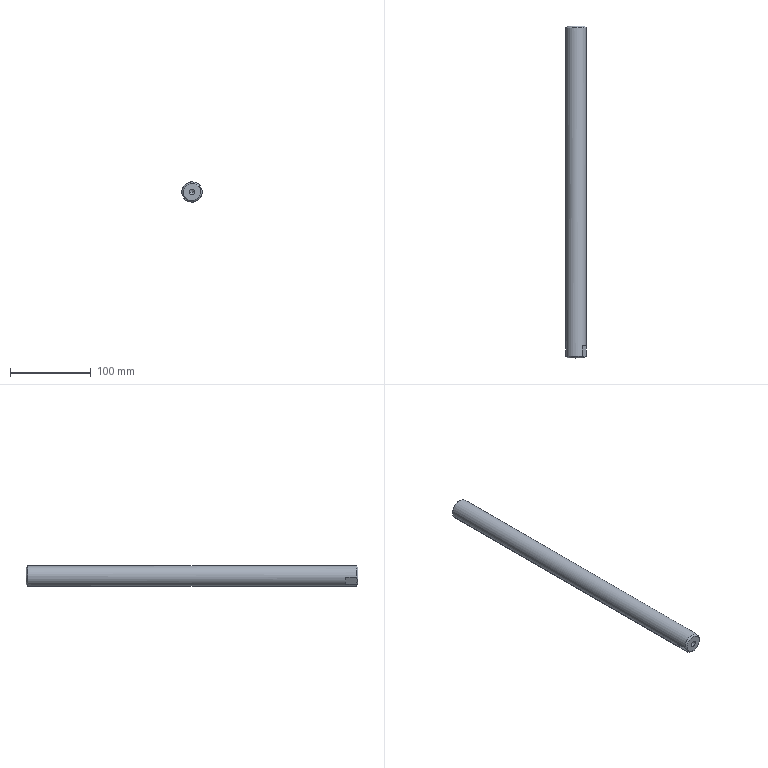Component | SolidWorks | PressingMechanism-08-2 | 1 solid | 16 faces | box 25 x 410 x 25 mm | volume 199952 mm3 | cone 6 | plane 6 | cylinder 4 | commonest cylinder face diameters 6.8 x2 25 x2
build123d program:
from build123d import *

# Parameters (mm, degrees)
SKETCH1_R             = 12.5
EXTRUDE1_DEPTH        = 410
M8_TAPPED_HOLE1_D     = 6.8
M8_TAPPED_HOLE1_DEPTH = 22.25
M8_TAPPED_HOLE1_TIP   = 2.043
CHAMFER1_SIZE         = 2
EXTRUDE2_DEPTH        = 411.381
EXTRUDE2_DEPTH_BACK   = 411.381
SKETCH6_W             = 15
SKETCH6_H             = 1


with BuildPart() as part:
    # Sketch1 → Extrude1 (new body)
    with BuildSketch(Plane(origin=(0, 0, 0), x_dir=(0, 0, -1), z_dir=(1, 0, 0))):
        with Locations(Location((0, 0, 0), (0, 0, 180))):
            Circle(SKETCH1_R)
    extrude(amount=EXTRUDE1_DEPTH)

    # M8 Tapped Hole1
    with Locations(Plane(origin=(410, 0, 0), x_dir=(0, 0, -1), z_dir=(1, 0, 0))):
        with Locations((0, 0)):
            Hole(M8_TAPPED_HOLE1_D / 2, depth=M8_TAPPED_HOLE1_DEPTH)
            with Locations((0, 0, -(M8_TAPPED_HOLE1_DEPTH + M8_TAPPED_HOLE1_TIP / 2))):  # 118° drill point
                Cone(0, M8_TAPPED_HOLE1_D / 2, M8_TAPPED_HOLE1_TIP, mode=Mode.SUBTRACT)

    # Chamfer1
    chamfer1_edges = [part.edges().sort_by_distance(p)[0] for p in [
        (0, 0, -12.5),
        (410, 0, -12.5),
    ]]
    chamfer(chamfer1_edges, length=CHAMFER1_SIZE)

    # Sketch6 → Extrude2 (cut, two sides: drawn at the far end of the back side and taken through both)
    with BuildSketch(Plane(origin=(0, 0, 0), x_dir=(1, 0, 0), z_dir=(0, 1, 0)).offset(-EXTRUDE2_DEPTH_BACK)):
        with Locations((402.5, 12)):
            Rectangle(SKETCH6_W, SKETCH6_H)
        with Locations((402.5, -12)):
            Rectangle(SKETCH6_W, SKETCH6_H)
    extrude(amount=EXTRUDE2_DEPTH + EXTRUDE2_DEPTH_BACK, mode=Mode.SUBTRACT)


solid = part.part

# Placed as in the assembly
solid = solid.moved(Location((-70, 354.5, 175), (0, 60.647, -90)))
STEP:
#1=CARTESIAN_POINT('',(-3.116,13.957,6.687));
#2=VERTEX_POINT('',#1);
#3=CARTESIAN_POINT('',(-2.396,13.957,7.092));
#4=VERTEX_POINT('',#3);
#5=CARTESIAN_POINT('',(-2.756,13.957,6.89));
#6=DIRECTION('',(0.,1.,-0.));
#7=DIRECTION('',(0.8716,0.,0.4902));
#8=AXIS2_PLACEMENT_3D('',#5,#6,#7);
#9=CIRCLE('',#8,0.4134);
#10=EDGE_CURVE('',#2,#4,#9,.T.);
#11=ORIENTED_EDGE('',*,*,#10,.F.);
#12=CARTESIAN_POINT('',(-3.185,13.878,6.649));
#13=VERTEX_POINT('',#12);
#14=CARTESIAN_POINT('',(-3.185,13.878,6.649));
#15=DIRECTION('',(-0.6163,-0.7071,-0.3466));
#16=VECTOR('',#15,39.37);
#17=LINE('',#14,#16);
#18=EDGE_CURVE('',#2,#13,#17,.T.);
#19=ORIENTED_EDGE('',*,*,#18,.T.);
#20=CARTESIAN_POINT('',(-2.327,13.878,7.131));
#21=VERTEX_POINT('',#20);
#22=CARTESIAN_POINT('',(-2.756,13.878,6.89));
#23=DIRECTION('',(-0.,-1.,0.));
#24=DIRECTION('',(0.8716,0.,0.4902));
#25=AXIS2_PLACEMENT_3D('',#22,#23,#24);
#26=CIRCLE('',#25,0.4921);
#27=EDGE_CURVE('',#21,#13,#26,.T.);
#28=ORIENTED_EDGE('',*,*,#27,.F.);
#29=CARTESIAN_POINT('',(-2.327,13.878,7.131));
#30=DIRECTION('',(0.6163,-0.7071,0.3466));
#31=VECTOR('',#30,39.37);
#32=LINE('',#29,#31);
#33=EDGE_CURVE('',#4,#21,#32,.T.);
#34=ORIENTED_EDGE('',*,*,#33,.F.);
#35=EDGE_LOOP('',(#11,#19,#28,#34));
#36=FACE_OUTER_BOUND('',#35,.T.);
#37=CARTESIAN_POINT('',(-2.756,13.878,6.89));
#38=DIRECTION('',(-0.,-1.,0.));
#39=DIRECTION('',(0.8716,0.,0.4902));
#40=AXIS2_PLACEMENT_3D('',#37,#38,#39);
#41=CONICAL_SURFACE('',#40,0.4921,0.7854);
#42=ADVANCED_FACE('',(#36),#41,.T.);
#43=CARTESIAN_POINT('',(-2.396,-2.185,7.092));
#44=VERTEX_POINT('',#43);
#45=CARTESIAN_POINT('',(-3.116,-2.185,6.687));
#46=VERTEX_POINT('',#45);
#47=CARTESIAN_POINT('',(-2.756,-2.185,6.89));
#48=DIRECTION('',(-0.,-1.,0.));
#49=DIRECTION('',(0.8716,0.,0.4902));
#50=AXIS2_PLACEMENT_3D('',#47,#48,#49);
#51=CIRCLE('',#50,0.4134);
#52=EDGE_CURVE('',#44,#46,#51,.T.);
#53=ORIENTED_EDGE('',*,*,#52,.F.);
#54=CARTESIAN_POINT('',(-2.361,-2.146,7.112));
#55=VERTEX_POINT('',#54);
#56=CARTESIAN_POINT('',(-2.396,-2.185,7.092));
#57=DIRECTION('',(0.6163,0.7071,0.3466));
#58=VECTOR('',#57,39.37);
#59=LINE('',#56,#58);
#60=EDGE_CURVE('',#44,#55,#59,.T.);
#61=ORIENTED_EDGE('',*,*,#60,.T.);
#62=CARTESIAN_POINT('',(-2.456,-2.106,7.28));
#63=VERTEX_POINT('',#62);
#64=CARTESIAN_POINT('',(-2.456,-2.106,7.28));
#65=CARTESIAN_POINT('',(-2.448,-2.112,7.266));
#66=CARTESIAN_POINT('',(-2.441,-2.118,7.253));
#67=CARTESIAN_POINT('',(-2.425,-2.128,7.225));
#68=CARTESIAN_POINT('',(-2.417,-2.132,7.211));
#69=CARTESIAN_POINT('',(-2.402,-2.139,7.183));
#70=CARTESIAN_POINT('',(-2.394,-2.141,7.169));
#71=CARTESIAN_POINT('',(-2.378,-2.145,7.141));
#72=CARTESIAN_POINT('',(-2.369,-2.146,7.126));
#73=CARTESIAN_POINT('',(-2.361,-2.146,7.112));
#74=B_SPLINE_CURVE_WITH_KNOTS('',3,(#64,#65,#66,#67,#68,#69,#70,#71,#72,#73),.UNSPECIFIED.,.F.,.F.,(4,2,2,2,4),(0.009607,0.01085,0.01209,0.01333,0.01458),.UNSPECIFIED.);
#75=EDGE_CURVE('',#63,#55,#74,.T.);
#76=ORIENTED_EDGE('',*,*,#75,.F.);
#77=CARTESIAN_POINT('',(-3.245,-2.106,6.836));
#78=VERTEX_POINT('',#77);
#79=CARTESIAN_POINT('',(-2.756,-2.106,6.89));
#80=DIRECTION('',(0.,1.,-0.));
#81=DIRECTION('',(0.8716,0.,0.4902));
#82=AXIS2_PLACEMENT_3D('',#79,#80,#81);
#83=CIRCLE('',#82,0.4921);
#84=EDGE_CURVE('',#78,#63,#83,.T.);
#85=ORIENTED_EDGE('',*,*,#84,.F.);
#86=CARTESIAN_POINT('',(-3.151,-2.146,6.668));
#87=VERTEX_POINT('',#86);
#88=CARTESIAN_POINT('',(-3.151,-2.146,6.668));
#89=CARTESIAN_POINT('',(-3.159,-2.146,6.682));
#90=CARTESIAN_POINT('',(-3.167,-2.145,6.697));
#91=CARTESIAN_POINT('',(-3.183,-2.141,6.725));
#92=CARTESIAN_POINT('',(-3.191,-2.139,6.74));
#93=CARTESIAN_POINT('',(-3.207,-2.132,6.768));
#94=CARTESIAN_POINT('',(-3.214,-2.128,6.781));
#95=CARTESIAN_POINT('',(-3.23,-2.118,6.809));
#96=CARTESIAN_POINT('',(-3.238,-2.112,6.823));
#97=CARTESIAN_POINT('',(-3.245,-2.106,6.836));
#98=B_SPLINE_CURVE_WITH_KNOTS('',3,(#88,#89,#90,#91,#92,#93,#94,#95,#96,#97),.UNSPECIFIED.,.F.,.F.,(4,2,2,2,4),(0.03511,0.03635,0.03759,0.03883,0.04007),.UNSPECIFIED.);
#99=EDGE_CURVE('',#87,#78,#98,.T.);
#100=ORIENTED_EDGE('',*,*,#99,.F.);
#101=CARTESIAN_POINT('',(-3.116,-2.185,6.687));
#102=DIRECTION('',(-0.6163,0.7071,-0.3466));
#103=VECTOR('',#102,39.37);
#104=LINE('',#101,#103);
#105=EDGE_CURVE('',#46,#87,#104,.T.);
#106=ORIENTED_EDGE('',*,*,#105,.F.);
#107=EDGE_LOOP('',(#53,#61,#76,#85,#100,#106));
#108=FACE_OUTER_BOUND('',#107,.T.);
#109=CARTESIAN_POINT('',(-2.756,-2.185,6.89));
#110=DIRECTION('',(0.,1.,-0.));
#111=DIRECTION('',(-0.8716,0.,-0.4902));
#112=AXIS2_PLACEMENT_3D('',#109,#110,#111);
#113=CONICAL_SURFACE('',#112,0.4134,0.7854);
#114=ADVANCED_FACE('',(#108),#113,.T.);
#115=CARTESIAN_POINT('',(-2.873,-1.309,6.824));
#116=VERTEX_POINT('',#115);
#117=CARTESIAN_POINT('',(-2.639,-1.309,6.955));
#118=VERTEX_POINT('',#117);
#119=CARTESIAN_POINT('',(-2.756,-1.309,6.89));
#120=DIRECTION('',(-0.,-1.,0.));
#121=DIRECTION('',(0.8716,0.,0.4902));
#122=AXIS2_PLACEMENT_3D('',#119,#120,#121);
#123=CIRCLE('',#122,0.1339);
#124=EDGE_CURVE('',#116,#118,#123,.T.);
#125=ORIENTED_EDGE('',*,*,#124,.F.);
#126=CARTESIAN_POINT('',(-2.873,-2.185,6.824));
#127=VERTEX_POINT('',#126);
#128=CARTESIAN_POINT('',(-2.873,-2.185,6.824));
#129=DIRECTION('',(-0.,-1.,0.));
#130=VECTOR('',#129,39.37);
#131=LINE('',#128,#130);
#132=EDGE_CURVE('',#116,#127,#131,.T.);
#133=ORIENTED_EDGE('',*,*,#132,.T.);
#134=CARTESIAN_POINT('',(-2.639,-2.185,6.955));
#135=VERTEX_POINT('',#134);
#136=CARTESIAN_POINT('',(-2.756,-2.185,6.89));
#137=DIRECTION('',(-0.,-1.,0.));
#138=DIRECTION('',(0.8716,0.,0.4902));
#139=AXIS2_PLACEMENT_3D('',#136,#137,#138);
#140=CIRCLE('',#139,0.1339);
#141=EDGE_CURVE('',#127,#135,#140,.T.);
#142=ORIENTED_EDGE('',*,*,#141,.T.);
#143=CARTESIAN_POINT('',(-2.639,-2.185,6.955));
#144=DIRECTION('',(-0.,-1.,0.));
#145=VECTOR('',#144,39.37);
#146=LINE('',#143,#145);
#147=EDGE_CURVE('',#118,#135,#146,.T.);
#148=ORIENTED_EDGE('',*,*,#147,.F.);
#149=EDGE_LOOP('',(#125,#133,#142,#148));
#150=FACE_OUTER_BOUND('',#149,.T.);
#151=CARTESIAN_POINT('',(-2.756,-2.185,6.89));
#152=DIRECTION('',(-0.,-1.,0.));
#153=DIRECTION('',(0.8716,0.,0.4902));
#154=AXIS2_PLACEMENT_3D('',#151,#152,#153);
#155=CYLINDRICAL_SURFACE('',#154,0.1339);
#156=ADVANCED_FACE('',(#150),#155,.F.);
#157=CARTESIAN_POINT('',(-2.756,-1.229,6.89));
#158=VERTEX_POINT('',#157);
#159=CARTESIAN_POINT('',(-2.639,-1.309,6.955));
#160=DIRECTION('',(0.7471,-0.515,0.4202));
#161=VECTOR('',#160,39.37);
#162=LINE('',#159,#161);
#163=EDGE_CURVE('',#158,#118,#162,.T.);
#164=ORIENTED_EDGE('',*,*,#163,.F.);
#165=CARTESIAN_POINT('',(-2.873,-1.309,6.824));
#166=DIRECTION('',(-0.7471,-0.515,-0.4202));
#167=VECTOR('',#166,39.37);
#168=LINE('',#165,#167);
#169=EDGE_CURVE('',#158,#116,#168,.T.);
#170=ORIENTED_EDGE('',*,*,#169,.T.);
#171=ORIENTED_EDGE('',*,*,#124,.T.);
#172=EDGE_LOOP('',(#164,#170,#171));
#173=FACE_OUTER_BOUND('',#172,.T.);
#174=CARTESIAN_POINT('',(-2.756,-1.309,6.89));
#175=DIRECTION('',(-0.,-1.,0.));
#176=DIRECTION('',(0.8716,0.,0.4902));
#177=AXIS2_PLACEMENT_3D('',#174,#175,#176);
#178=CONICAL_SURFACE('',#177,0.1339,1.03);
#179=ADVANCED_FACE('',(#173),#178,.F.);
#180=CARTESIAN_POINT('',(-2.456,-1.594,7.28));
#181=VERTEX_POINT('',#180);
#182=CARTESIAN_POINT('',(-2.327,-1.594,7.131));
#183=VERTEX_POINT('',#182);
#184=CARTESIAN_POINT('',(-2.756,-1.594,6.89));
#185=DIRECTION('',(0.,1.,-0.));
#186=DIRECTION('',(-0.8716,-0.,-0.4902));
#187=AXIS2_PLACEMENT_3D('',#184,#185,#186);
#188=CIRCLE('',#187,0.4921);
#189=EDGE_CURVE('',#181,#183,#188,.T.);
#190=ORIENTED_EDGE('',*,*,#189,.T.);
#191=CARTESIAN_POINT('',(-2.327,-2.185,7.131));
#192=DIRECTION('',(0.,1.,-0.));
#193=VECTOR('',#192,39.37);
#194=LINE('',#191,#193);
#195=EDGE_CURVE('',#183,#21,#194,.T.);
#196=ORIENTED_EDGE('',*,*,#195,.T.);
#197=ORIENTED_EDGE('',*,*,#27,.T.);
#198=CARTESIAN_POINT('',(-3.185,-1.594,6.649));
#199=VERTEX_POINT('',#198);
#200=CARTESIAN_POINT('',(-3.185,-2.185,6.649));
#201=DIRECTION('',(0.,1.,-0.));
#202=VECTOR('',#201,39.37);
#203=LINE('',#200,#202);
#204=EDGE_CURVE('',#199,#13,#203,.T.);
#205=ORIENTED_EDGE('',*,*,#204,.F.);
#206=CARTESIAN_POINT('',(-3.245,-1.594,6.836));
#207=VERTEX_POINT('',#206);
#208=CARTESIAN_POINT('',(-2.756,-1.594,6.89));
#209=DIRECTION('',(0.,1.,-0.));
#210=DIRECTION('',(-0.8716,-0.,-0.4902));
#211=AXIS2_PLACEMENT_3D('',#208,#209,#210);
#212=CIRCLE('',#211,0.4921);
#213=EDGE_CURVE('',#199,#207,#212,.T.);
#214=ORIENTED_EDGE('',*,*,#213,.T.);
#215=CARTESIAN_POINT('',(-3.245,-2.185,6.836));
#216=DIRECTION('',(-0.,-1.,0.));
#217=VECTOR('',#216,39.37);
#218=LINE('',#215,#217);
#219=EDGE_CURVE('',#207,#78,#218,.T.);
#220=ORIENTED_EDGE('',*,*,#219,.T.);
#221=ORIENTED_EDGE('',*,*,#84,.T.);
#222=CARTESIAN_POINT('',(-2.456,-2.185,7.28));
#223=DIRECTION('',(0.,1.,-0.));
#224=VECTOR('',#223,39.37);
#225=LINE('',#222,#224);
#226=EDGE_CURVE('',#63,#181,#225,.T.);
#227=ORIENTED_EDGE('',*,*,#226,.T.);
#228=EDGE_LOOP('',(#190,#196,#197,#205,#214,#220,#221,#227));
#229=FACE_OUTER_BOUND('',#228,.T.);
#230=CARTESIAN_POINT('',(-2.756,-2.185,6.89));
#231=DIRECTION('',(0.,1.,-0.));
#232=DIRECTION('',(-0.8716,-0.,-0.4902));
#233=AXIS2_PLACEMENT_3D('',#230,#231,#232);
#234=CYLINDRICAL_SURFACE('',#233,0.4921);
#235=ADVANCED_FACE('',(#229),#234,.T.);
#236=ORIENTED_EDGE('',*,*,#195,.F.);
#237=CARTESIAN_POINT('',(-2.267,-1.594,6.944));
#238=VERTEX_POINT('',#237);
#239=CARTESIAN_POINT('',(-2.756,-1.594,6.89));
#240=DIRECTION('',(0.,1.,-0.));
#241=DIRECTION('',(-0.8716,-0.,-0.4902));
#242=AXIS2_PLACEMENT_3D('',#239,#240,#241);
#243=CIRCLE('',#242,0.4921);
#244=EDGE_CURVE('',#183,#238,#243,.T.);
#245=ORIENTED_EDGE('',*,*,#244,.T.);
#246=CARTESIAN_POINT('',(-2.267,-2.106,6.944));
#247=VERTEX_POINT('',#246);
#248=CARTESIAN_POINT('',(-2.267,-2.185,6.944));
#249=DIRECTION('',(-0.,-1.,0.));
#250=VECTOR('',#249,39.37);
#251=LINE('',#248,#250);
#252=EDGE_CURVE('',#238,#247,#251,.T.);
#253=ORIENTED_EDGE('',*,*,#252,.T.);
#254=CARTESIAN_POINT('',(-3.056,-2.106,6.5));
#255=VERTEX_POINT('',#254);
#256=CARTESIAN_POINT('',(-2.756,-2.106,6.89));
#257=DIRECTION('',(0.,1.,-0.));
#258=DIRECTION('',(0.8716,0.,0.4902));
#259=AXIS2_PLACEMENT_3D('',#256,#257,#258);
#260=CIRCLE('',#259,0.4921);
#261=EDGE_CURVE('',#247,#255,#260,.T.);
#262=ORIENTED_EDGE('',*,*,#261,.T.);
#263=CARTESIAN_POINT('',(-3.056,-1.594,6.5));
#264=VERTEX_POINT('',#263);
#265=CARTESIAN_POINT('',(-3.056,-2.185,6.5));
#266=DIRECTION('',(0.,1.,-0.));
#267=VECTOR('',#266,39.37);
#268=LINE('',#265,#267);
#269=EDGE_CURVE('',#255,#264,#268,.T.);
#270=ORIENTED_EDGE('',*,*,#269,.T.);
#271=CARTESIAN_POINT('',(-2.756,-1.594,6.89));
#272=DIRECTION('',(0.,1.,-0.));
#273=DIRECTION('',(-0.8716,-0.,-0.4902));
#274=AXIS2_PLACEMENT_3D('',#271,#272,#273);
#275=CIRCLE('',#274,0.4921);
#276=EDGE_CURVE('',#264,#199,#275,.T.);
#277=ORIENTED_EDGE('',*,*,#276,.T.);
#278=ORIENTED_EDGE('',*,*,#204,.T.);
#279=CARTESIAN_POINT('',(-2.756,13.878,6.89));
#280=DIRECTION('',(-0.,-1.,0.));
#281=DIRECTION('',(0.8716,0.,0.4902));
#282=AXIS2_PLACEMENT_3D('',#279,#280,#281);
#283=CIRCLE('',#282,0.4921);
#284=EDGE_CURVE('',#13,#21,#283,.T.);
#285=ORIENTED_EDGE('',*,*,#284,.T.);
#286=EDGE_LOOP('',(#236,#245,#253,#262,#270,#277,#278,#285));
#287=FACE_OUTER_BOUND('',#286,.T.);
#288=CARTESIAN_POINT('',(-2.756,-2.185,6.89));
#289=DIRECTION('',(0.,1.,-0.));
#290=DIRECTION('',(-0.8716,-0.,-0.4902));
#291=AXIS2_PLACEMENT_3D('',#288,#289,#290);
#292=CYLINDRICAL_SURFACE('',#291,0.4921);
#293=ADVANCED_FACE('',(#287),#292,.T.);
#294=CARTESIAN_POINT('',(-2.756,-2.185,6.89));
#295=DIRECTION('',(-0.,-1.,0.));
#296=DIRECTION('',(0.8716,0.,0.4902));
#297=AXIS2_PLACEMENT_3D('',#294,#295,#296);
#298=CIRCLE('',#297,0.4134);
#299=EDGE_CURVE('',#46,#44,#298,.T.);
#300=ORIENTED_EDGE('',*,*,#299,.T.);
#301=ORIENTED_EDGE('',*,*,#52,.T.);
#302=EDGE_LOOP('',(#300,#301));
#303=FACE_OUTER_BOUND('',#302,.T.);
#304=CARTESIAN_POINT('',(-2.756,-2.185,6.89));
#305=DIRECTION('',(-0.,-1.,0.));
#306=DIRECTION('',(0.8716,0.,0.4902));
#307=AXIS2_PLACEMENT_3D('',#304,#305,#306);
#308=CIRCLE('',#307,0.1339);
#309=EDGE_CURVE('',#135,#127,#308,.T.);
#310=ORIENTED_EDGE('',*,*,#309,.F.);
#311=ORIENTED_EDGE('',*,*,#141,.F.);
#312=EDGE_LOOP('',(#310,#311));
#313=FACE_BOUND('',#312,.T.);
#314=CARTESIAN_POINT('',(-2.756,-2.185,6.89));
#315=DIRECTION('',(-0.,-1.,0.));
#316=DIRECTION('',(0.8716,0.,0.4902));
#317=AXIS2_PLACEMENT_3D('',#314,#315,#316);
#318=PLANE('',#317);
#319=ADVANCED_FACE('',(#303,#313),#318,.T.);
#320=CARTESIAN_POINT('',(-2.756,13.957,6.89));
#321=DIRECTION('',(0.,1.,-0.));
#322=DIRECTION('',(0.8716,0.,0.4902));
#323=AXIS2_PLACEMENT_3D('',#320,#321,#322);
#324=CIRCLE('',#323,0.4134);
#325=EDGE_CURVE('',#4,#2,#324,.T.);
#326=ORIENTED_EDGE('',*,*,#325,.T.);
#327=ORIENTED_EDGE('',*,*,#10,.T.);
#328=EDGE_LOOP('',(#326,#327));
#329=FACE_OUTER_BOUND('',#328,.T.);
#330=CARTESIAN_POINT('',(-2.756,13.957,6.89));
#331=DIRECTION('',(-0.,-1.,0.));
#332=DIRECTION('',(0.8716,0.,0.4902));
#333=AXIS2_PLACEMENT_3D('',#330,#331,#332);
#334=PLANE('',#333);
#335=ADVANCED_FACE('',(#329),#334,.F.);
#336=ORIENTED_EDGE('',*,*,#169,.F.);
#337=ORIENTED_EDGE('',*,*,#163,.T.);
#338=CARTESIAN_POINT('',(-2.756,-1.309,6.89));
#339=DIRECTION('',(-0.,-1.,0.));
#340=DIRECTION('',(0.8716,0.,0.4902));
#341=AXIS2_PLACEMENT_3D('',#338,#339,#340);
#342=CIRCLE('',#341,0.1339);
#343=EDGE_CURVE('',#118,#116,#342,.T.);
#344=ORIENTED_EDGE('',*,*,#343,.T.);
#345=EDGE_LOOP('',(#336,#337,#344));
#346=FACE_OUTER_BOUND('',#345,.T.);
#347=CARTESIAN_POINT('',(-2.756,-1.309,6.89));
#348=DIRECTION('',(-0.,-1.,0.));
#349=DIRECTION('',(0.8716,0.,0.4902));
#350=AXIS2_PLACEMENT_3D('',#347,#348,#349);
#351=CONICAL_SURFACE('',#350,0.1339,1.03);
#352=ADVANCED_FACE('',(#346),#351,.F.);
#353=ORIENTED_EDGE('',*,*,#132,.F.);
#354=ORIENTED_EDGE('',*,*,#343,.F.);
#355=ORIENTED_EDGE('',*,*,#147,.T.);
#356=ORIENTED_EDGE('',*,*,#309,.T.);
#357=EDGE_LOOP('',(#353,#354,#355,#356));
#358=FACE_OUTER_BOUND('',#357,.T.);
#359=CARTESIAN_POINT('',(-2.756,-2.185,6.89));
#360=DIRECTION('',(-0.,-1.,0.));
#361=DIRECTION('',(0.8716,0.,0.4902));
#362=AXIS2_PLACEMENT_3D('',#359,#360,#361);
#363=CYLINDRICAL_SURFACE('',#362,0.1339);
#364=ADVANCED_FACE('',(#358),#363,.F.);
#365=ORIENTED_EDGE('',*,*,#60,.F.);
#366=ORIENTED_EDGE('',*,*,#299,.F.);
#367=ORIENTED_EDGE('',*,*,#105,.T.);
#368=CARTESIAN_POINT('',(-3.056,-2.106,6.5));
#369=CARTESIAN_POINT('',(-3.063,-2.112,6.513));
#370=CARTESIAN_POINT('',(-3.071,-2.118,6.526));
#371=CARTESIAN_POINT('',(-3.086,-2.127,6.554));
#372=CARTESIAN_POINT('',(-3.094,-2.132,6.568));
#373=CARTESIAN_POINT('',(-3.118,-2.142,6.61));
#374=CARTESIAN_POINT('',(-3.134,-2.146,6.639));
#375=CARTESIAN_POINT('',(-3.151,-2.146,6.668));
#376=B_SPLINE_CURVE_WITH_KNOTS('',3,(#368,#369,#370,#371,#372,#373,#374,#375),.UNSPECIFIED.,.F.,.F.,(4,2,2,4),(0.03014,0.03138,0.03262,0.03511),.UNSPECIFIED.);
#377=EDGE_CURVE('',#255,#87,#376,.T.);
#378=ORIENTED_EDGE('',*,*,#377,.F.);
#379=ORIENTED_EDGE('',*,*,#261,.F.);
#380=CARTESIAN_POINT('',(-2.361,-2.146,7.112));
#381=CARTESIAN_POINT('',(-2.345,-2.146,7.083));
#382=CARTESIAN_POINT('',(-2.329,-2.142,7.054));
#383=CARTESIAN_POINT('',(-2.305,-2.132,7.012));
#384=CARTESIAN_POINT('',(-2.297,-2.127,6.998));
#385=CARTESIAN_POINT('',(-2.282,-2.118,6.97));
#386=CARTESIAN_POINT('',(-2.274,-2.112,6.957));
#387=CARTESIAN_POINT('',(-2.267,-2.106,6.944));
#388=B_SPLINE_CURVE_WITH_KNOTS('',3,(#380,#381,#382,#383,#384,#385,#386,#387),.UNSPECIFIED.,.F.,.F.,(4,2,2,4),(0.01458,0.01707,0.01831,0.01956),.UNSPECIFIED.);
#389=EDGE_CURVE('',#55,#247,#388,.T.);
#390=ORIENTED_EDGE('',*,*,#389,.F.);
#391=EDGE_LOOP('',(#365,#366,#367,#378,#379,#390));
#392=FACE_OUTER_BOUND('',#391,.T.);
#393=CARTESIAN_POINT('',(-2.756,-2.185,6.89));
#394=DIRECTION('',(0.,1.,-0.));
#395=DIRECTION('',(-0.8716,0.,-0.4902));
#396=AXIS2_PLACEMENT_3D('',#393,#394,#395);
#397=CONICAL_SURFACE('',#396,0.4134,0.7854);
#398=ADVANCED_FACE('',(#392),#397,.T.);
#399=ORIENTED_EDGE('',*,*,#18,.F.);
#400=ORIENTED_EDGE('',*,*,#325,.F.);
#401=ORIENTED_EDGE('',*,*,#33,.T.);
#402=ORIENTED_EDGE('',*,*,#284,.F.);
#403=EDGE_LOOP('',(#399,#400,#401,#402));
#404=FACE_OUTER_BOUND('',#403,.T.);
#405=CARTESIAN_POINT('',(-2.756,13.878,6.89));
#406=DIRECTION('',(-0.,-1.,0.));
#407=DIRECTION('',(0.8716,0.,0.4902));
#408=AXIS2_PLACEMENT_3D('',#405,#406,#407);
#409=CONICAL_SURFACE('',#408,0.4921,0.7854);
#410=ADVANCED_FACE('',(#404),#409,.T.);
#411=CARTESIAN_POINT('',(-2.12,-1.594,6.683));
#412=DIRECTION('',(-0.4902,0.,0.8716));
#413=VECTOR('',#412,39.37);
#414=LINE('',#411,#413);
#415=EDGE_CURVE('',#238,#181,#414,.T.);
#416=ORIENTED_EDGE('',*,*,#415,.F.);
#417=ORIENTED_EDGE('',*,*,#244,.F.);
#418=ORIENTED_EDGE('',*,*,#189,.F.);
#419=EDGE_LOOP('',(#416,#417,#418));
#420=FACE_OUTER_BOUND('',#419,.T.);
#421=CARTESIAN_POINT('',(-2.12,-1.594,6.683));
#422=DIRECTION('',(0.,1.,-0.));
#423=DIRECTION('',(-0.8716,-0.,-0.4902));
#424=AXIS2_PLACEMENT_3D('',#421,#422,#423);
#425=PLANE('',#424);
#426=ADVANCED_FACE('',(#420),#425,.F.);
#427=ORIENTED_EDGE('',*,*,#75,.T.);
#428=ORIENTED_EDGE('',*,*,#389,.T.);
#429=ORIENTED_EDGE('',*,*,#252,.F.);
#430=ORIENTED_EDGE('',*,*,#415,.T.);
#431=ORIENTED_EDGE('',*,*,#226,.F.);
#432=EDGE_LOOP('',(#427,#428,#429,#430,#431));
#433=FACE_OUTER_BOUND('',#432,.T.);
#434=CARTESIAN_POINT('',(-2.12,-2.185,6.683));
#435=DIRECTION('',(-0.8716,-0.,-0.4902));
#436=DIRECTION('',(0.,-1.,0.));
#437=AXIS2_PLACEMENT_3D('',#434,#435,#436);
#438=PLANE('',#437);
#439=ADVANCED_FACE('',(#433),#438,.F.);
#440=ORIENTED_EDGE('',*,*,#276,.F.);
#441=CARTESIAN_POINT('',(-2.909,-1.594,6.239));
#442=DIRECTION('',(-0.4902,0.,0.8716));
#443=VECTOR('',#442,39.37);
#444=LINE('',#441,#443);
#445=EDGE_CURVE('',#264,#207,#444,.T.);
#446=ORIENTED_EDGE('',*,*,#445,.T.);
#447=ORIENTED_EDGE('',*,*,#213,.F.);
#448=EDGE_LOOP('',(#440,#446,#447));
#449=FACE_OUTER_BOUND('',#448,.T.);
#450=CARTESIAN_POINT('',(-2.909,-1.594,6.239));
#451=DIRECTION('',(0.,1.,-0.));
#452=DIRECTION('',(-0.8716,-0.,-0.4902));
#453=AXIS2_PLACEMENT_3D('',#450,#451,#452);
#454=PLANE('',#453);
#455=ADVANCED_FACE('',(#449),#454,.F.);
#456=ORIENTED_EDGE('',*,*,#377,.T.);
#457=ORIENTED_EDGE('',*,*,#99,.T.);
#458=ORIENTED_EDGE('',*,*,#219,.F.);
#459=ORIENTED_EDGE('',*,*,#445,.F.);
#460=ORIENTED_EDGE('',*,*,#269,.F.);
#461=EDGE_LOOP('',(#456,#457,#458,#459,#460));
#462=FACE_OUTER_BOUND('',#461,.T.);
#463=CARTESIAN_POINT('',(-2.909,-2.185,6.239));
#464=DIRECTION('',(0.8716,0.,0.4902));
#465=DIRECTION('',(0.,1.,-0.));
#466=AXIS2_PLACEMENT_3D('',#463,#464,#465);
#467=PLANE('',#466);
#468=ADVANCED_FACE('',(#462),#467,.F.);
#469=CLOSED_SHELL('',(#42,#114,#156,#179,#235,#293,#319,#335,#352,#364,#398,#410,#426,#439,#455,#468));
#470=MANIFOLD_SOLID_BREP('',#469);
#471=CARTESIAN_POINT('',(0.,0.,0.));
#472=DIRECTION('',(0.,0.,1.));
#473=DIRECTION('',(1.,0.,0.));
#474=AXIS2_PLACEMENT_3D('',#471,#472,#473);
#475=(LENGTH_UNIT()NAMED_UNIT(*)SI_UNIT($,.METRE.));
#476=LENGTH_MEASURE_WITH_UNIT(LENGTH_MEASURE(0.0254),#475);
#477=DIMENSIONAL_EXPONENTS(1.,0.,0.,0.,0.,0.,0.);
#478=(CONVERSION_BASED_UNIT('',#476)LENGTH_UNIT()NAMED_UNIT(#477));
#479=UNCERTAINTY_MEASURE_WITH_UNIT(LENGTH_MEASURE(0.00001),#478,'','');
#480=(NAMED_UNIT(*)PLANE_ANGLE_UNIT()SI_UNIT($,.RADIAN.));
#481=(NAMED_UNIT(*)SI_UNIT($,.STERADIAN.)SOLID_ANGLE_UNIT());
#482=(GEOMETRIC_REPRESENTATION_CONTEXT(3)GLOBAL_UNCERTAINTY_ASSIGNED_CONTEXT((#479))GLOBAL_UNIT_ASSIGNED_CONTEXT((#478,#480,#481))REPRESENTATION_CONTEXT('',''));
#483=ADVANCED_BREP_SHAPE_REPRESENTATION('',(#470,#474),#482);
#484=COLOUR_RGB('',0.7922,0.8196,0.9333);
#485=FILL_AREA_STYLE_COLOUR('',#484);
#486=FILL_AREA_STYLE('',(#485));
#487=SURFACE_STYLE_FILL_AREA(#486);
#488=SURFACE_SIDE_STYLE('',(#487));
#489=SURFACE_STYLE_USAGE(.BOTH.,#488);
#490=PRESENTATION_STYLE_ASSIGNMENT((#489));
#491=STYLED_ITEM('',(#490),#470);
#492=PRESENTATION_LAYER_ASSIGNMENT('','',(#491));
#493=(LENGTH_UNIT()NAMED_UNIT(*)SI_UNIT($,.METRE.));
#494=LENGTH_MEASURE_WITH_UNIT(LENGTH_MEASURE(0.0254),#493);
#495=DIMENSIONAL_EXPONENTS(1.,0.,0.,0.,0.,0.,0.);
#496=(CONVERSION_BASED_UNIT('',#494)LENGTH_UNIT()NAMED_UNIT(#495));
#497=UNCERTAINTY_MEASURE_WITH_UNIT(LENGTH_MEASURE(0.00001),#496,'','');
#498=(NAMED_UNIT(*)PLANE_ANGLE_UNIT()SI_UNIT($,.RADIAN.));
#499=(NAMED_UNIT(*)SI_UNIT($,.STERADIAN.)SOLID_ANGLE_UNIT());
#500=(GEOMETRIC_REPRESENTATION_CONTEXT(3)GLOBAL_UNCERTAINTY_ASSIGNED_CONTEXT((#497))GLOBAL_UNIT_ASSIGNED_CONTEXT((#496,#498,#499))REPRESENTATION_CONTEXT('',''));
#501=MECHANICAL_DESIGN_GEOMETRIC_PRESENTATION_REPRESENTATION('',(#491),#500);